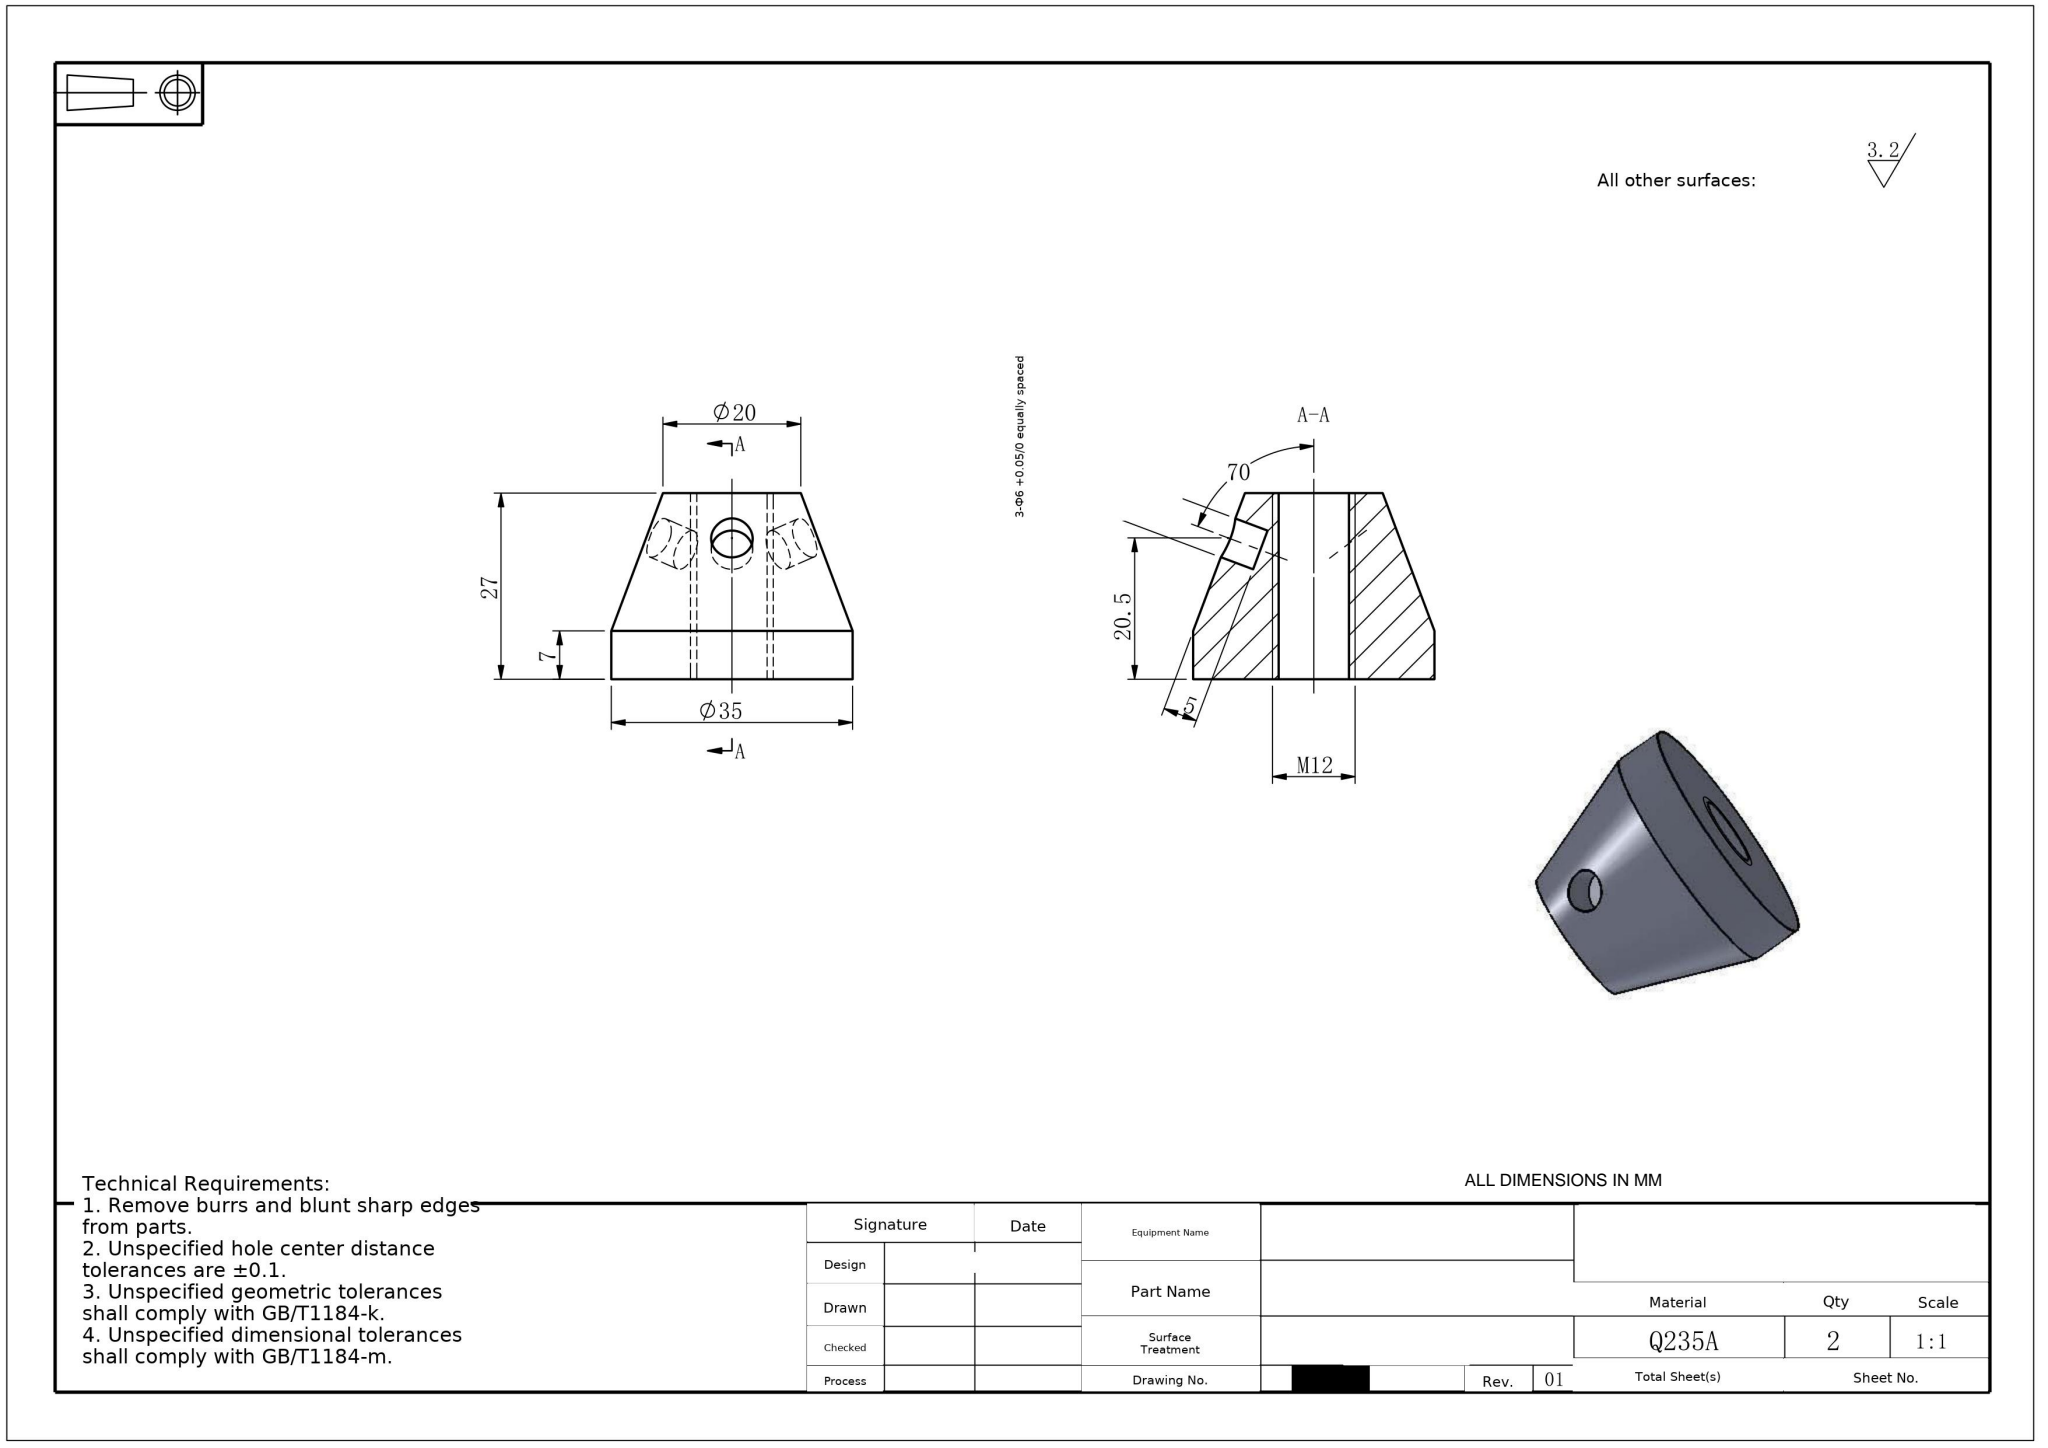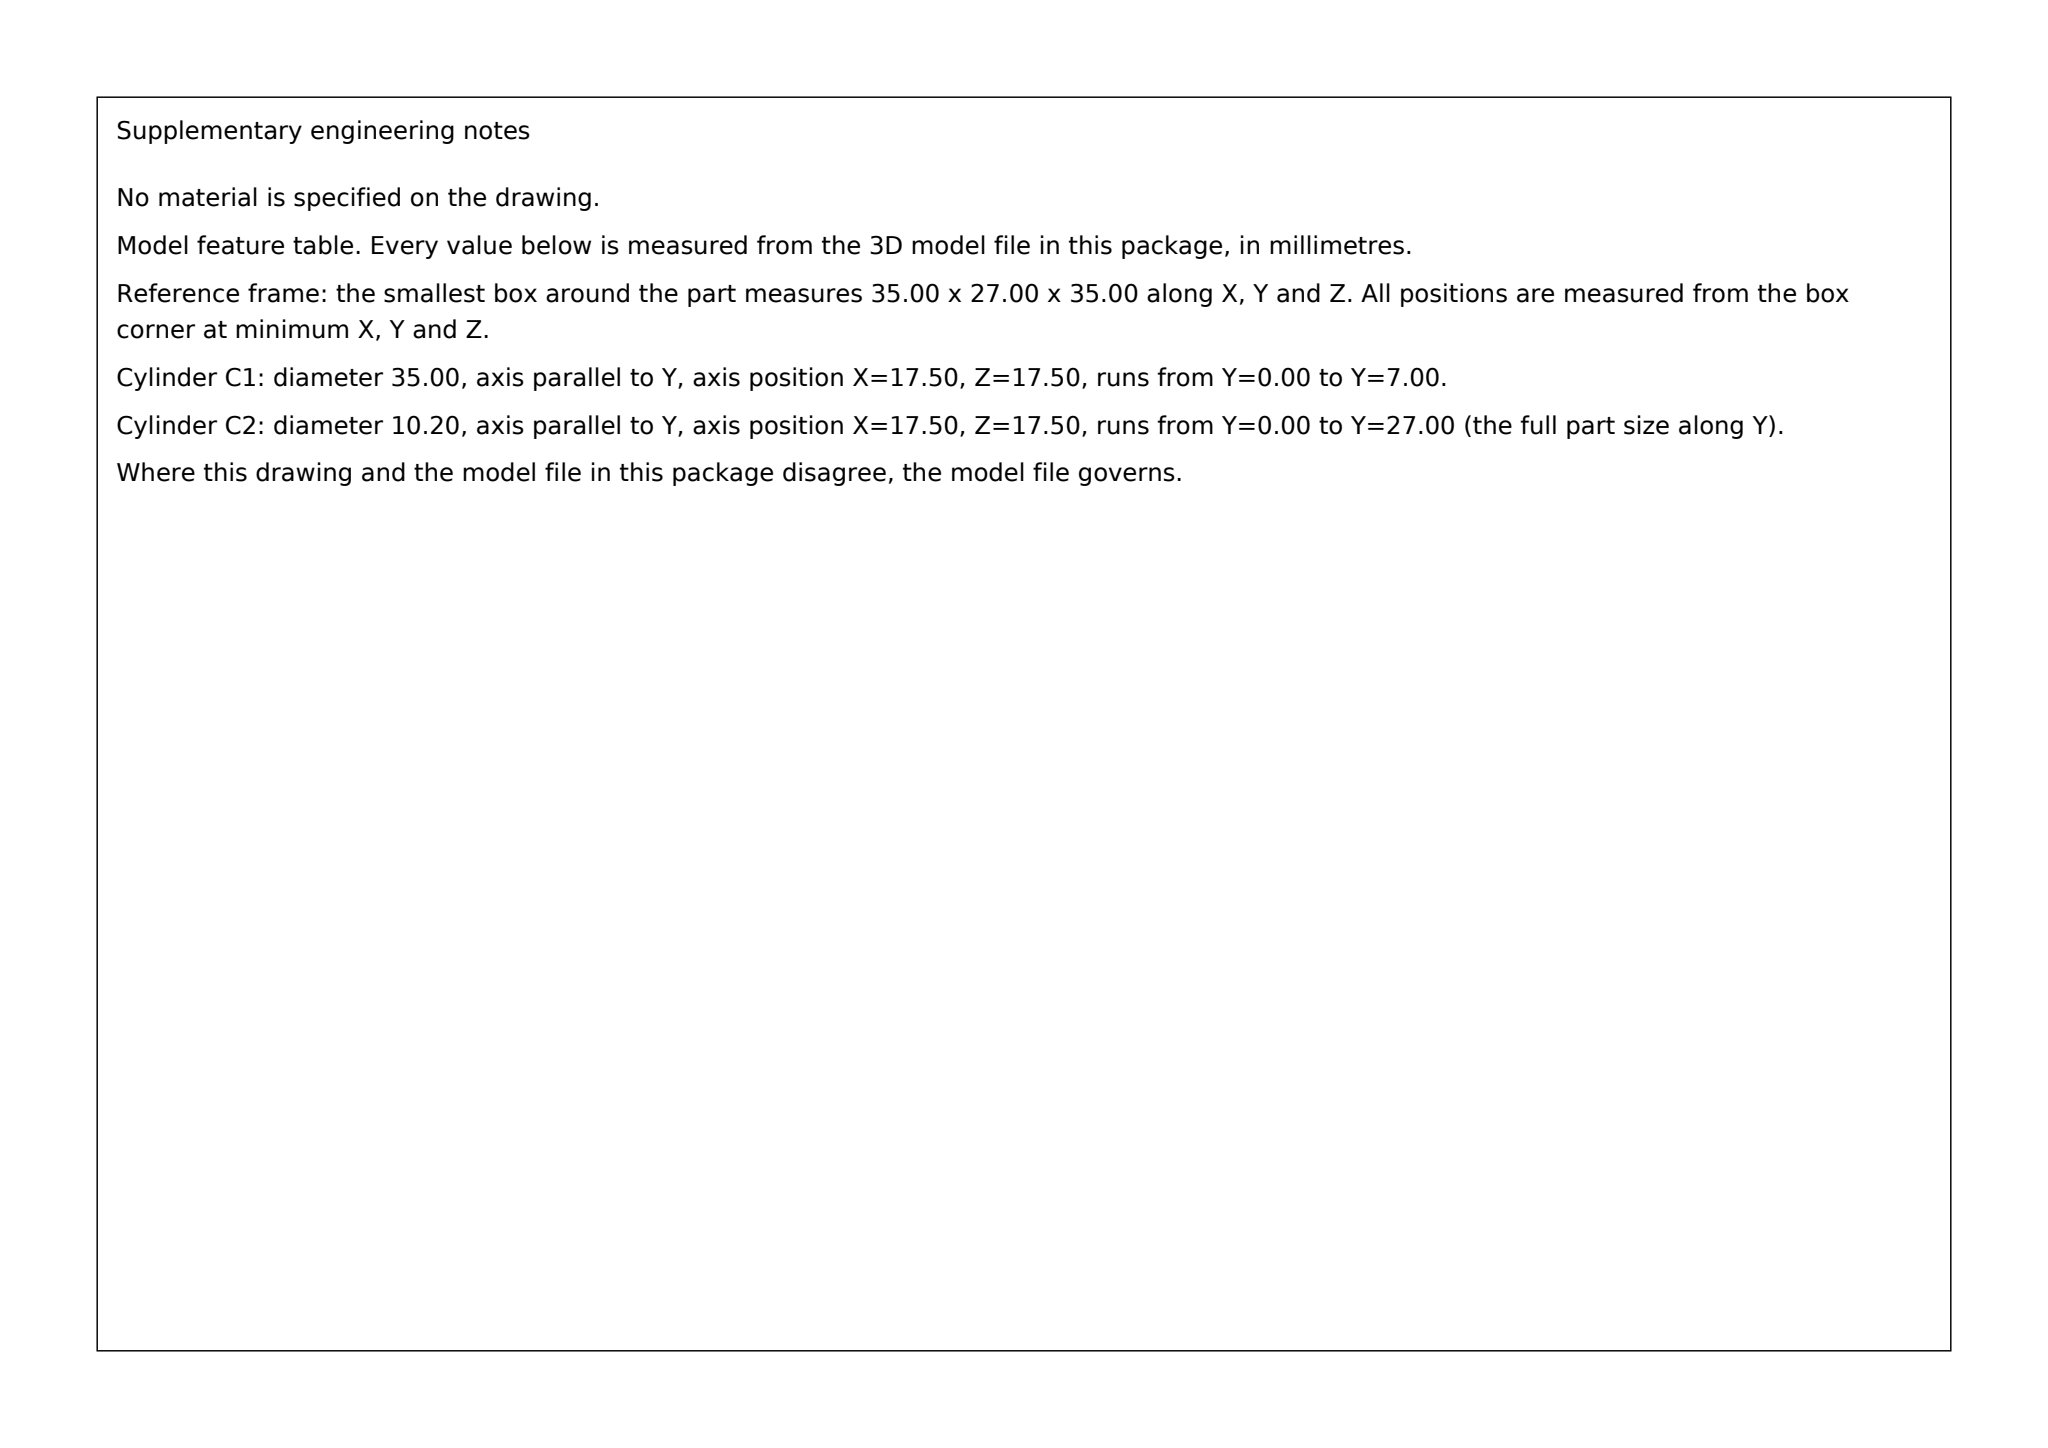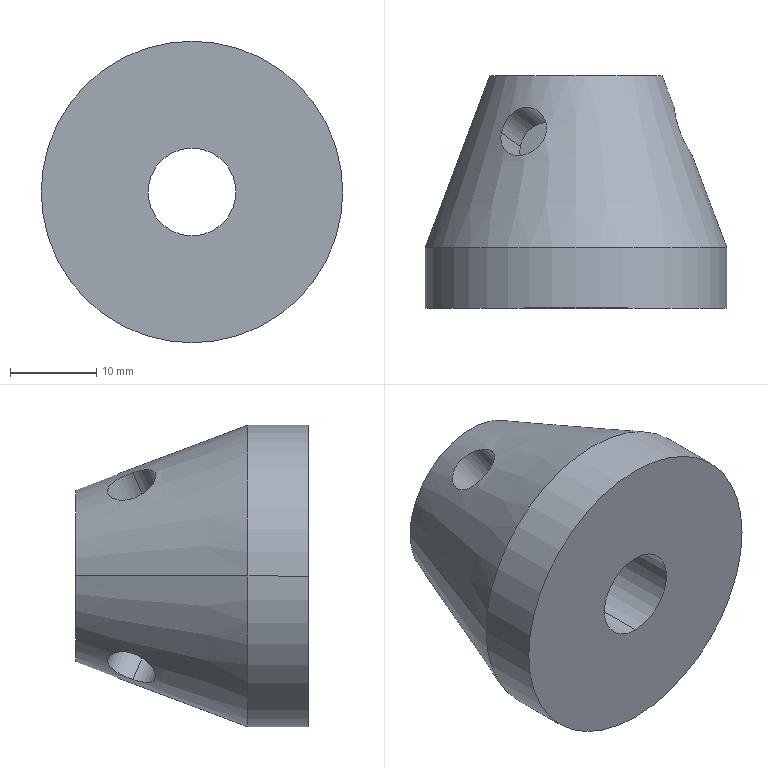Part | SolidWorks | mm | 1 solid | 17 faces | box 35 x 27 x 35 mm | volume 16285 mm3 | cylinder 10 | plane 5 | cone 2 | commonest cylinder face diameters 6 x6 10.2 x2 35 x2
STEP:
#1=CARTESIAN_POINT('',(-48.239,6.094,-8.217));
#2=VERTEX_POINT('',#1);
#3=CARTESIAN_POINT('',(-53.435,6.094,-5.217));
#4=VERTEX_POINT('',#3);
#5=CARTESIAN_POINT('',(-50.837,6.094,-6.717));
#6=DIRECTION('',(-0.4682,0.3511,-0.8109));
#7=DIRECTION('',(0.1756,0.9363,0.3041));
#8=AXIS2_PLACEMENT_3D('',#5,#6,#7);
#9=CIRCLE('',#8,3.);
#10=EDGE_CURVE('',#2,#4,#9,.T.);
#11=ORIENTED_EDGE('',*,*,#10,.F.);
#12=CARTESIAN_POINT('',(-50.42,7.729,-11.993));
#13=VERTEX_POINT('',#12);
#14=CARTESIAN_POINT('',(-48.239,6.094,-8.217));
#15=DIRECTION('',(-0.4682,0.3511,-0.8109));
#16=VECTOR('',#15,1000.);
#17=LINE('',#14,#16);
#18=EDGE_CURVE('',#2,#13,#17,.T.);
#19=ORIENTED_EDGE('',*,*,#18,.T.);
#20=CARTESIAN_POINT('',(-55.616,7.729,-8.993));
#21=VERTEX_POINT('',#20);
#22=CARTESIAN_POINT('',(-55.616,7.729,-8.993));
#23=CARTESIAN_POINT('',(-55.651,7.545,-9.055));
#24=CARTESIAN_POINT('',(-55.672,7.362,-9.13));
#25=CARTESIAN_POINT('',(-55.683,7.01,-9.302));
#26=CARTESIAN_POINT('',(-55.673,6.837,-9.4));
#27=CARTESIAN_POINT('',(-55.622,6.508,-9.614));
#28=CARTESIAN_POINT('',(-55.581,6.354,-9.728));
#29=CARTESIAN_POINT('',(-55.469,6.065,-9.969));
#30=CARTESIAN_POINT('',(-55.397,5.928,-10.097));
#31=CARTESIAN_POINT('',(-55.227,5.685,-10.354));
#32=CARTESIAN_POINT('',(-55.128,5.576,-10.484));
#33=CARTESIAN_POINT('',(-54.902,5.386,-10.746));
#34=CARTESIAN_POINT('',(-54.775,5.304,-10.876));
#35=CARTESIAN_POINT('',(-54.501,5.173,-11.127));
#36=CARTESIAN_POINT('',(-54.352,5.123,-11.25));
#37=CARTESIAN_POINT('',(-54.038,5.057,-11.479));
#38=CARTESIAN_POINT('',(-53.874,5.041,-11.586));
#39=CARTESIAN_POINT('',(-53.533,5.041,-11.782));
#40=CARTESIAN_POINT('',(-53.355,5.058,-11.873));
#41=CARTESIAN_POINT('',(-53.002,5.124,-12.028));
#42=CARTESIAN_POINT('',(-52.824,5.174,-12.096));
#43=CARTESIAN_POINT('',(-52.467,5.306,-12.208));
#44=CARTESIAN_POINT('',(-52.292,5.386,-12.252));
#45=CARTESIAN_POINT('',(-51.955,5.576,-12.316));
#46=CARTESIAN_POINT('',(-51.79,5.686,-12.337));
#47=CARTESIAN_POINT('',(-51.481,5.931,-12.356));
#48=CARTESIAN_POINT('',(-51.338,6.065,-12.355));
#49=CARTESIAN_POINT('',(-51.073,6.354,-12.331));
#50=CARTESIAN_POINT('',(-50.952,6.512,-12.308));
#51=CARTESIAN_POINT('',(-50.743,6.838,-12.246));
#52=CARTESIAN_POINT('',(-50.654,7.008,-12.206));
#53=CARTESIAN_POINT('',(-50.509,7.364,-12.11));
#54=CARTESIAN_POINT('',(-50.455,7.547,-12.055));
#55=CARTESIAN_POINT('',(-50.42,7.729,-11.993));
#56=B_SPLINE_CURVE_WITH_KNOTS('',3,(#22,#23,#24,#25,#26,#27,#28,#29,#30,#31,#32,#33,#34,#35,#36,#37,#38,#39,#40,#41,#42,#43,#44,#45,#46,#47,#48,#49,#50,#51,#52,#53,#54,#55),.UNSPECIFIED.,.F.,.F.,(4,2,2,2,2,2,2,2,2,2,2,2,2,2,2,2,4),(0.01489,0.01548,0.01607,0.01665,0.01724,0.01783,0.01842,0.01901,0.01959,0.02018,0.02077,0.02136,0.02195,0.02253,0.02312,0.02371,0.0243),.UNSPECIFIED.);
#57=EDGE_CURVE('',#21,#13,#56,.T.);
#58=ORIENTED_EDGE('',*,*,#57,.F.);
#59=CARTESIAN_POINT('',(-53.435,6.094,-5.217));
#60=DIRECTION('',(-0.4682,0.3511,-0.8109));
#61=VECTOR('',#60,1000.);
#62=LINE('',#59,#61);
#63=EDGE_CURVE('',#4,#21,#62,.T.);
#64=ORIENTED_EDGE('',*,*,#63,.F.);
#65=EDGE_LOOP('',(#11,#19,#58,#64));
#66=FACE_OUTER_BOUND('',#65,.T.);
#67=CARTESIAN_POINT('',(-50.837,6.094,-6.717));
#68=DIRECTION('',(-0.4682,0.3511,-0.8109));
#69=DIRECTION('',(-0.866,0.,0.5));
#70=AXIS2_PLACEMENT_3D('',#67,#68,#69);
#71=CYLINDRICAL_SURFACE('',#70,3.);
#72=ADVANCED_FACE('',(#66),#71,.F.);
#73=CARTESIAN_POINT('',(-53.435,6.094,5.217));
#74=VERTEX_POINT('',#73);
#75=CARTESIAN_POINT('',(-48.239,6.094,8.217));
#76=VERTEX_POINT('',#75);
#77=CARTESIAN_POINT('',(-50.837,6.094,6.717));
#78=DIRECTION('',(-0.4682,0.3511,0.8109));
#79=DIRECTION('',(0.1756,0.9363,-0.3041));
#80=AXIS2_PLACEMENT_3D('',#77,#78,#79);
#81=CIRCLE('',#80,3.);
#82=EDGE_CURVE('',#74,#76,#81,.T.);
#83=ORIENTED_EDGE('',*,*,#82,.F.);
#84=CARTESIAN_POINT('',(-55.616,7.729,8.993));
#85=VERTEX_POINT('',#84);
#86=CARTESIAN_POINT('',(-53.435,6.094,5.217));
#87=DIRECTION('',(-0.4682,0.3511,0.8109));
#88=VECTOR('',#87,1000.);
#89=LINE('',#86,#88);
#90=EDGE_CURVE('',#74,#85,#89,.T.);
#91=ORIENTED_EDGE('',*,*,#90,.T.);
#92=CARTESIAN_POINT('',(-50.42,7.729,11.993));
#93=VERTEX_POINT('',#92);
#94=CARTESIAN_POINT('',(-50.42,7.729,11.993));
#95=CARTESIAN_POINT('',(-50.455,7.546,12.055));
#96=CARTESIAN_POINT('',(-50.51,7.362,12.111));
#97=CARTESIAN_POINT('',(-50.654,7.009,12.206));
#98=CARTESIAN_POINT('',(-50.743,6.838,12.246));
#99=CARTESIAN_POINT('',(-50.954,6.508,12.309));
#100=CARTESIAN_POINT('',(-51.074,6.353,12.331));
#101=CARTESIAN_POINT('',(-51.338,6.064,12.355));
#102=CARTESIAN_POINT('',(-51.484,5.928,12.356));
#103=CARTESIAN_POINT('',(-51.794,5.684,12.337));
#104=CARTESIAN_POINT('',(-51.956,5.576,12.316));
#105=CARTESIAN_POINT('',(-52.294,5.386,12.252));
#106=CARTESIAN_POINT('',(-52.471,5.304,12.207));
#107=CARTESIAN_POINT('',(-52.824,5.174,12.095));
#108=CARTESIAN_POINT('',(-53.002,5.124,12.028));
#109=CARTESIAN_POINT('',(-53.358,5.057,11.871));
#110=CARTESIAN_POINT('',(-53.535,5.041,11.781));
#111=CARTESIAN_POINT('',(-53.874,5.041,11.585));
#112=CARTESIAN_POINT('',(-54.04,5.057,11.478));
#113=CARTESIAN_POINT('',(-54.355,5.124,11.247));
#114=CARTESIAN_POINT('',(-54.502,5.174,11.127));
#115=CARTESIAN_POINT('',(-54.775,5.304,10.876));
#116=CARTESIAN_POINT('',(-54.902,5.386,10.745));
#117=CARTESIAN_POINT('',(-55.128,5.576,10.485));
#118=CARTESIAN_POINT('',(-55.227,5.684,10.355));
#119=CARTESIAN_POINT('',(-55.398,5.929,10.096));
#120=CARTESIAN_POINT('',(-55.469,6.065,9.969));
#121=CARTESIAN_POINT('',(-55.581,6.354,9.729));
#122=CARTESIAN_POINT('',(-55.622,6.508,9.614));
#123=CARTESIAN_POINT('',(-55.673,6.839,9.399));
#124=CARTESIAN_POINT('',(-55.683,7.009,9.302));
#125=CARTESIAN_POINT('',(-55.672,7.361,9.131));
#126=CARTESIAN_POINT('',(-55.651,7.545,9.055));
#127=CARTESIAN_POINT('',(-55.616,7.729,8.993));
#128=B_SPLINE_CURVE_WITH_KNOTS('',3,(#94,#95,#96,#97,#98,#99,#100,#101,#102,#103,#104,#105,#106,#107,#108,#109,#110,#111,#112,#113,#114,#115,#116,#117,#118,#119,#120,#121,#122,#123,#124,#125,#126,#127),.UNSPECIFIED.,.F.,.F.,(4,2,2,2,2,2,2,2,2,2,2,2,2,2,2,2,4),(0.008823,0.009411,0.009999,0.01059,0.01117,0.01176,0.01235,0.01294,0.01353,0.01411,0.0147,0.01529,0.01588,0.01647,0.01705,0.01764,0.01823),.UNSPECIFIED.);
#129=EDGE_CURVE('',#93,#85,#128,.T.);
#130=ORIENTED_EDGE('',*,*,#129,.F.);
#131=CARTESIAN_POINT('',(-48.239,6.094,8.217));
#132=DIRECTION('',(-0.4682,0.3511,0.8109));
#133=VECTOR('',#132,1000.);
#134=LINE('',#131,#133);
#135=EDGE_CURVE('',#76,#93,#134,.T.);
#136=ORIENTED_EDGE('',*,*,#135,.F.);
#137=EDGE_LOOP('',(#83,#91,#130,#136));
#138=FACE_OUTER_BOUND('',#137,.T.);
#139=CARTESIAN_POINT('',(-50.837,6.094,6.717));
#140=DIRECTION('',(-0.4682,0.3511,0.8109));
#141=DIRECTION('',(0.866,0.,0.5));
#142=AXIS2_PLACEMENT_3D('',#139,#140,#141);
#143=CYLINDRICAL_SURFACE('',#142,3.);
#144=ADVANCED_FACE('',(#138),#143,.F.);
#145=CARTESIAN_POINT('',(-38.15,3.285,0.));
#146=VERTEX_POINT('',#145);
#147=CARTESIAN_POINT('',(-40.257,8.903,0.));
#148=VERTEX_POINT('',#147);
#149=CARTESIAN_POINT('',(-39.203,6.094,0.));
#150=DIRECTION('',(0.9363,0.3511,-0.));
#151=DIRECTION('',(-0.3511,0.9363,0.));
#152=AXIS2_PLACEMENT_3D('',#149,#150,#151);
#153=CIRCLE('',#152,3.);
#154=EDGE_CURVE('',#146,#148,#153,.T.);
#155=ORIENTED_EDGE('',*,*,#154,.F.);
#156=CARTESIAN_POINT('',(-33.468,5.041,0.));
#157=VERTEX_POINT('',#156);
#158=CARTESIAN_POINT('',(-38.15,3.285,0.));
#159=DIRECTION('',(0.9363,0.3511,-0.));
#160=VECTOR('',#159,1000.);
#161=LINE('',#158,#160);
#162=EDGE_CURVE('',#146,#157,#161,.T.);
#163=ORIENTED_EDGE('',*,*,#162,.T.);
#164=CARTESIAN_POINT('',(-35.575,10.659,0.));
#165=VERTEX_POINT('',#164);
#166=CARTESIAN_POINT('',(-35.575,10.659,0.));
#167=CARTESIAN_POINT('',(-35.575,10.659,-0.1967));
#168=CARTESIAN_POINT('',(-35.573,10.639,-0.3918));
#169=CARTESIAN_POINT('',(-35.563,10.56,-0.7784));
#170=CARTESIAN_POINT('',(-35.556,10.501,-0.969));
#171=CARTESIAN_POINT('',(-35.535,10.349,-1.33));
#172=CARTESIAN_POINT('',(-35.521,10.255,-1.503));
#173=CARTESIAN_POINT('',(-35.485,10.035,-1.831));
#174=CARTESIAN_POINT('',(-35.463,9.911,-1.982));
#175=CARTESIAN_POINT('',(-35.41,9.637,-2.258));
#176=CARTESIAN_POINT('',(-35.377,9.485,-2.384));
#177=CARTESIAN_POINT('',(-35.302,9.166,-2.602));
#178=CARTESIAN_POINT('',(-35.258,8.998,-2.694));
#179=CARTESIAN_POINT('',(-35.159,8.648,-2.845));
#180=CARTESIAN_POINT('',(-35.103,8.465,-2.903));
#181=CARTESIAN_POINT('',(-34.981,8.1,-2.98));
#182=CARTESIAN_POINT('',(-34.915,7.917,-3.));
#183=CARTESIAN_POINT('',(-34.772,7.547,-3.));
#184=CARTESIAN_POINT('',(-34.697,7.365,-2.981));
#185=CARTESIAN_POINT('',(-34.543,7.012,-2.904));
#186=CARTESIAN_POINT('',(-34.462,6.839,-2.847));
#187=CARTESIAN_POINT('',(-34.303,6.51,-2.696));
#188=CARTESIAN_POINT('',(-34.225,6.356,-2.604));
#189=CARTESIAN_POINT('',(-34.071,6.066,-2.387));
#190=CARTESIAN_POINT('',(-33.996,5.93,-2.26));
#191=CARTESIAN_POINT('',(-33.859,5.685,-1.984));
#192=CARTESIAN_POINT('',(-33.795,5.575,-1.831));
#193=CARTESIAN_POINT('',(-33.681,5.384,-1.503));
#194=CARTESIAN_POINT('',(-33.632,5.304,-1.331));
#195=CARTESIAN_POINT('',(-33.552,5.174,-0.9692));
#196=CARTESIAN_POINT('',(-33.521,5.124,-0.7778));
#197=CARTESIAN_POINT('',(-33.479,5.057,-0.3924));
#198=CARTESIAN_POINT('',(-33.468,5.041,-0.1974));
#199=CARTESIAN_POINT('',(-33.468,5.041,0.));
#200=B_SPLINE_CURVE_WITH_KNOTS('',3,(#166,#167,#168,#169,#170,#171,#172,#173,#174,#175,#176,#177,#178,#179,#180,#181,#182,#183,#184,#185,#186,#187,#188,#189,#190,#191,#192,#193,#194,#195,#196,#197,#198,#199),.UNSPECIFIED.,.F.,.F.,(4,2,2,2,2,2,2,2,2,2,2,2,2,2,2,2,4),(0.01126,0.01185,0.01244,0.01303,0.01362,0.01421,0.01479,0.01538,0.01597,0.01656,0.01715,0.01773,0.01832,0.01891,0.0195,0.02009,0.02068),.UNSPECIFIED.);
#201=EDGE_CURVE('',#165,#157,#200,.T.);
#202=ORIENTED_EDGE('',*,*,#201,.F.);
#203=CARTESIAN_POINT('',(-40.257,8.903,0.));
#204=DIRECTION('',(0.9363,0.3511,-0.));
#205=VECTOR('',#204,1000.);
#206=LINE('',#203,#205);
#207=EDGE_CURVE('',#148,#165,#206,.T.);
#208=ORIENTED_EDGE('',*,*,#207,.F.);
#209=EDGE_LOOP('',(#155,#163,#202,#208));
#210=FACE_OUTER_BOUND('',#209,.T.);
#211=CARTESIAN_POINT('',(-39.203,6.094,0.));
#212=DIRECTION('',(0.9363,0.3511,-0.));
#213=DIRECTION('',(-0.3511,0.9363,0.));
#214=AXIS2_PLACEMENT_3D('',#211,#212,#213);
#215=CYLINDRICAL_SURFACE('',#214,3.);
#216=ADVANCED_FACE('',(#210),#215,.F.);
#217=CARTESIAN_POINT('',(-46.959,14.35,5.1));
#218=VERTEX_POINT('',#217);
#219=CARTESIAN_POINT('',(-46.959,14.35,-5.1));
#220=VERTEX_POINT('',#219);
#221=CARTESIAN_POINT('',(-46.959,14.35,0.));
#222=DIRECTION('',(0.,-1.,0.));
#223=DIRECTION('',(0.,0.,-1.));
#224=AXIS2_PLACEMENT_3D('',#221,#222,#223);
#225=CIRCLE('',#224,5.1);
#226=EDGE_CURVE('',#218,#220,#225,.T.);
#227=ORIENTED_EDGE('',*,*,#226,.F.);
#228=CARTESIAN_POINT('',(-46.959,-12.65,5.1));
#229=VERTEX_POINT('',#228);
#230=CARTESIAN_POINT('',(-46.959,-12.65,5.1));
#231=DIRECTION('',(0.,-1.,0.));
#232=VECTOR('',#231,1000.);
#233=LINE('',#230,#232);
#234=EDGE_CURVE('',#218,#229,#233,.T.);
#235=ORIENTED_EDGE('',*,*,#234,.T.);
#236=CARTESIAN_POINT('',(-46.959,-12.65,-5.1));
#237=VERTEX_POINT('',#236);
#238=CARTESIAN_POINT('',(-46.959,-12.65,0.));
#239=DIRECTION('',(0.,-1.,0.));
#240=DIRECTION('',(0.,0.,-1.));
#241=AXIS2_PLACEMENT_3D('',#238,#239,#240);
#242=CIRCLE('',#241,5.1);
#243=EDGE_CURVE('',#229,#237,#242,.T.);
#244=ORIENTED_EDGE('',*,*,#243,.T.);
#245=CARTESIAN_POINT('',(-46.959,-12.65,-5.1));
#246=DIRECTION('',(0.,-1.,0.));
#247=VECTOR('',#246,1000.);
#248=LINE('',#245,#247);
#249=EDGE_CURVE('',#220,#237,#248,.T.);
#250=ORIENTED_EDGE('',*,*,#249,.F.);
#251=EDGE_LOOP('',(#227,#235,#244,#250));
#252=FACE_OUTER_BOUND('',#251,.T.);
#253=CARTESIAN_POINT('',(-46.959,-12.65,0.));
#254=DIRECTION('',(0.,-1.,0.));
#255=DIRECTION('',(0.,0.,-1.));
#256=AXIS2_PLACEMENT_3D('',#253,#254,#255);
#257=CYLINDRICAL_SURFACE('',#256,5.1);
#258=ADVANCED_FACE('',(#252),#257,.F.);
#259=CARTESIAN_POINT('',(-64.459,-12.65,0.));
#260=VERTEX_POINT('',#259);
#261=CARTESIAN_POINT('',(-29.459,-12.65,0.));
#262=VERTEX_POINT('',#261);
#263=CARTESIAN_POINT('',(-46.959,-12.65,0.));
#264=DIRECTION('',(0.,1.,0.));
#265=DIRECTION('',(-1.,0.,0.));
#266=AXIS2_PLACEMENT_3D('',#263,#264,#265);
#267=CIRCLE('',#266,17.5);
#268=EDGE_CURVE('',#260,#262,#267,.T.);
#269=ORIENTED_EDGE('',*,*,#268,.T.);
#270=CARTESIAN_POINT('',(-29.459,-5.65,0.));
#271=VERTEX_POINT('',#270);
#272=CARTESIAN_POINT('',(-29.459,14.35,0.));
#273=DIRECTION('',(0.,1.,0.));
#274=VECTOR('',#273,1000.);
#275=LINE('',#272,#274);
#276=EDGE_CURVE('',#262,#271,#275,.T.);
#277=ORIENTED_EDGE('',*,*,#276,.T.);
#278=CARTESIAN_POINT('',(-64.459,-5.65,0.));
#279=VERTEX_POINT('',#278);
#280=CARTESIAN_POINT('',(-46.959,-5.65,0.));
#281=DIRECTION('',(0.,1.,0.));
#282=DIRECTION('',(-1.,0.,0.));
#283=AXIS2_PLACEMENT_3D('',#280,#281,#282);
#284=CIRCLE('',#283,17.5);
#285=EDGE_CURVE('',#279,#271,#284,.T.);
#286=ORIENTED_EDGE('',*,*,#285,.F.);
#287=CARTESIAN_POINT('',(-64.459,14.35,0.));
#288=DIRECTION('',(0.,1.,0.));
#289=VECTOR('',#288,1000.);
#290=LINE('',#287,#289);
#291=EDGE_CURVE('',#260,#279,#290,.T.);
#292=ORIENTED_EDGE('',*,*,#291,.F.);
#293=EDGE_LOOP('',(#269,#277,#286,#292));
#294=FACE_OUTER_BOUND('',#293,.T.);
#295=CARTESIAN_POINT('',(-46.959,14.35,0.));
#296=DIRECTION('',(0.,1.,0.));
#297=DIRECTION('',(-1.,0.,0.));
#298=AXIS2_PLACEMENT_3D('',#295,#296,#297);
#299=CYLINDRICAL_SURFACE('',#298,17.5);
#300=ADVANCED_FACE('',(#294),#299,.T.);
#301=ORIENTED_EDGE('',*,*,#129,.T.);
#302=CARTESIAN_POINT('',(-55.616,7.729,8.993));
#303=CARTESIAN_POINT('',(-55.544,8.098,8.87));
#304=CARTESIAN_POINT('',(-55.413,8.474,8.802));
#305=CARTESIAN_POINT('',(-55.144,8.997,8.786));
#306=CARTESIAN_POINT('',(-55.04,9.167,8.795));
#307=CARTESIAN_POINT('',(-54.813,9.487,8.839));
#308=CARTESIAN_POINT('',(-54.69,9.636,8.873));
#309=CARTESIAN_POINT('',(-54.423,9.911,8.965));
#310=CARTESIAN_POINT('',(-54.279,10.037,9.022));
#311=CARTESIAN_POINT('',(-53.98,10.255,9.154));
#312=CARTESIAN_POINT('',(-53.825,10.349,9.228));
#313=CARTESIAN_POINT('',(-53.335,10.579,9.474));
#314=CARTESIAN_POINT('',(-52.993,10.659,9.662));
#315=CARTESIAN_POINT('',(-52.478,10.658,9.959));
#316=CARTESIAN_POINT('',(-52.31,10.638,10.058));
#317=CARTESIAN_POINT('',(-51.982,10.56,10.259));
#318=CARTESIAN_POINT('',(-51.82,10.501,10.361));
#319=CARTESIAN_POINT('',(-51.517,10.348,10.561));
#320=CARTESIAN_POINT('',(-51.375,10.254,10.658));
#321=CARTESIAN_POINT('',(-51.11,10.034,10.853));
#322=CARTESIAN_POINT('',(-50.989,9.909,10.948));
#323=CARTESIAN_POINT('',(-50.777,9.634,11.132));
#324=CARTESIAN_POINT('',(-50.685,9.484,11.223));
#325=CARTESIAN_POINT('',(-50.533,9.163,11.398));
#326=CARTESIAN_POINT('',(-50.475,8.995,11.482));
#327=CARTESIAN_POINT('',(-50.395,8.646,11.643));
#328=CARTESIAN_POINT('',(-50.373,8.463,11.72));
#329=CARTESIAN_POINT('',(-50.368,8.097,11.865));
#330=CARTESIAN_POINT('',(-50.384,7.913,11.932));
#331=CARTESIAN_POINT('',(-50.42,7.729,11.993));
#332=B_SPLINE_CURVE_WITH_KNOTS('',3,(#302,#303,#304,#305,#306,#307,#308,#309,#310,#311,#312,#313,#314,#315,#316,#317,#318,#319,#320,#321,#322,#323,#324,#325,#326,#327,#328,#329,#330,#331),.UNSPECIFIED.,.F.,.F.,(4,2,2,2,2,2,2,2,2,2,2,2,2,2,4),(0.01823,0.0194,0.01999,0.02058,0.02117,0.02176,0.02293,0.02352,0.02411,0.0247,0.02529,0.02587,0.02646,0.02705,0.02764),.UNSPECIFIED.);
#333=EDGE_CURVE('',#85,#93,#332,.T.);
#334=ORIENTED_EDGE('',*,*,#333,.T.);
#335=EDGE_LOOP('',(#301,#334));
#336=FACE_BOUND('',#335,.T.);
#337=CARTESIAN_POINT('',(-56.959,14.35,0.));
#338=VERTEX_POINT('',#337);
#339=CARTESIAN_POINT('',(-36.959,14.35,0.));
#340=VERTEX_POINT('',#339);
#341=CARTESIAN_POINT('',(-46.959,14.35,0.));
#342=DIRECTION('',(0.,1.,0.));
#343=DIRECTION('',(-1.,0.,0.));
#344=AXIS2_PLACEMENT_3D('',#341,#342,#343);
#345=CIRCLE('',#344,10.);
#346=EDGE_CURVE('',#338,#340,#345,.T.);
#347=ORIENTED_EDGE('',*,*,#346,.F.);
#348=CARTESIAN_POINT('',(-64.459,-5.65,0.));
#349=DIRECTION('',(-0.3511,-0.9363,0.));
#350=VECTOR('',#349,1000.);
#351=LINE('',#348,#350);
#352=EDGE_CURVE('',#338,#279,#351,.T.);
#353=ORIENTED_EDGE('',*,*,#352,.T.);
#354=ORIENTED_EDGE('',*,*,#285,.T.);
#355=CARTESIAN_POINT('',(-29.459,-5.65,0.));
#356=DIRECTION('',(0.3511,-0.9363,0.));
#357=VECTOR('',#356,1000.);
#358=LINE('',#355,#357);
#359=EDGE_CURVE('',#157,#271,#358,.T.);
#360=ORIENTED_EDGE('',*,*,#359,.F.);
#361=CARTESIAN_POINT('',(-33.468,5.041,0.));
#362=CARTESIAN_POINT('',(-33.468,5.041,0.1974));
#363=CARTESIAN_POINT('',(-33.479,5.058,0.3959));
#364=CARTESIAN_POINT('',(-33.521,5.124,0.7802));
#365=CARTESIAN_POINT('',(-33.552,5.174,0.9689));
#366=CARTESIAN_POINT('',(-33.633,5.305,1.334));
#367=CARTESIAN_POINT('',(-33.682,5.386,1.507));
#368=CARTESIAN_POINT('',(-33.795,5.576,1.831));
#369=CARTESIAN_POINT('',(-33.859,5.687,1.985));
#370=CARTESIAN_POINT('',(-33.997,5.931,2.261));
#371=CARTESIAN_POINT('',(-34.07,6.064,2.385));
#372=CARTESIAN_POINT('',(-34.224,6.355,2.603));
#373=CARTESIAN_POINT('',(-34.304,6.512,2.697));
#374=CARTESIAN_POINT('',(-34.462,6.838,2.846));
#375=CARTESIAN_POINT('',(-34.541,7.008,2.903));
#376=CARTESIAN_POINT('',(-34.697,7.365,2.981));
#377=CARTESIAN_POINT('',(-34.772,7.547,3.));
#378=CARTESIAN_POINT('',(-34.913,7.912,3.));
#379=CARTESIAN_POINT('',(-34.98,8.099,2.98));
#380=CARTESIAN_POINT('',(-35.103,8.466,2.903));
#381=CARTESIAN_POINT('',(-35.158,8.646,2.846));
#382=CARTESIAN_POINT('',(-35.258,8.995,2.696));
#383=CARTESIAN_POINT('',(-35.302,9.167,2.601));
#384=CARTESIAN_POINT('',(-35.377,9.485,2.384));
#385=CARTESIAN_POINT('',(-35.409,9.634,2.26));
#386=CARTESIAN_POINT('',(-35.491,10.049,1.843));
#387=CARTESIAN_POINT('',(-35.524,10.272,1.514));
#388=CARTESIAN_POINT('',(-35.556,10.502,0.9677));
#389=CARTESIAN_POINT('',(-35.563,10.56,0.7805));
#390=CARTESIAN_POINT('',(-35.573,10.638,0.3962));
#391=CARTESIAN_POINT('',(-35.575,10.659,0.1967));
#392=CARTESIAN_POINT('',(-35.575,10.659,0.));
#393=B_SPLINE_CURVE_WITH_KNOTS('',3,(#361,#362,#363,#364,#365,#366,#367,#368,#369,#370,#371,#372,#373,#374,#375,#376,#377,#378,#379,#380,#381,#382,#383,#384,#385,#386,#387,#388,#389,#390,#391,#392),.UNSPECIFIED.,.F.,.F.,(4,2,2,2,2,2,2,2,2,2,2,2,2,2,2,4),(0.001855,0.002443,0.003031,0.003619,0.004207,0.004796,0.005384,0.005972,0.00656,0.007148,0.007736,0.008324,0.008912,0.01009,0.01068,0.01126),.UNSPECIFIED.);
#394=EDGE_CURVE('',#157,#165,#393,.T.);
#395=ORIENTED_EDGE('',*,*,#394,.T.);
#396=CARTESIAN_POINT('',(-29.459,-5.65,0.));
#397=DIRECTION('',(0.3511,-0.9363,0.));
#398=VECTOR('',#397,1000.);
#399=LINE('',#396,#398);
#400=EDGE_CURVE('',#340,#165,#399,.T.);
#401=ORIENTED_EDGE('',*,*,#400,.F.);
#402=EDGE_LOOP('',(#347,#353,#354,#360,#395,#401));
#403=FACE_OUTER_BOUND('',#402,.T.);
#404=CARTESIAN_POINT('',(-46.959,-5.65,0.));
#405=DIRECTION('',(-0.,-1.,0.));
#406=DIRECTION('',(1.,-0.,0.));
#407=AXIS2_PLACEMENT_3D('',#404,#405,#406);
#408=CONICAL_SURFACE('',#407,17.5,0.3588);
#409=ADVANCED_FACE('',(#336,#403),#408,.T.);
#410=CARTESIAN_POINT('',(-46.959,14.35,0.));
#411=DIRECTION('',(0.,-1.,0.));
#412=DIRECTION('',(0.,0.,-1.));
#413=AXIS2_PLACEMENT_3D('',#410,#411,#412);
#414=CIRCLE('',#413,5.1);
#415=EDGE_CURVE('',#220,#218,#414,.T.);
#416=ORIENTED_EDGE('',*,*,#415,.T.);
#417=ORIENTED_EDGE('',*,*,#226,.T.);
#418=EDGE_LOOP('',(#416,#417));
#419=FACE_BOUND('',#418,.T.);
#420=CARTESIAN_POINT('',(-46.959,14.35,0.));
#421=DIRECTION('',(0.,1.,0.));
#422=DIRECTION('',(-1.,0.,0.));
#423=AXIS2_PLACEMENT_3D('',#420,#421,#422);
#424=CIRCLE('',#423,10.);
#425=EDGE_CURVE('',#340,#338,#424,.T.);
#426=ORIENTED_EDGE('',*,*,#425,.T.);
#427=ORIENTED_EDGE('',*,*,#346,.T.);
#428=EDGE_LOOP('',(#426,#427));
#429=FACE_OUTER_BOUND('',#428,.T.);
#430=CARTESIAN_POINT('',(-46.959,14.35,0.));
#431=DIRECTION('',(-0.,-1.,0.));
#432=DIRECTION('',(1.,-0.,0.));
#433=AXIS2_PLACEMENT_3D('',#430,#431,#432);
#434=PLANE('',#433);
#435=ADVANCED_FACE('',(#419,#429),#434,.F.);
#436=ORIENTED_EDGE('',*,*,#352,.F.);
#437=ORIENTED_EDGE('',*,*,#425,.F.);
#438=ORIENTED_EDGE('',*,*,#400,.T.);
#439=ORIENTED_EDGE('',*,*,#201,.T.);
#440=ORIENTED_EDGE('',*,*,#359,.T.);
#441=CARTESIAN_POINT('',(-46.959,-5.65,0.));
#442=DIRECTION('',(0.,1.,0.));
#443=DIRECTION('',(-1.,0.,0.));
#444=AXIS2_PLACEMENT_3D('',#441,#442,#443);
#445=CIRCLE('',#444,17.5);
#446=EDGE_CURVE('',#271,#279,#445,.T.);
#447=ORIENTED_EDGE('',*,*,#446,.T.);
#448=EDGE_LOOP('',(#436,#437,#438,#439,#440,#447));
#449=FACE_OUTER_BOUND('',#448,.T.);
#450=ORIENTED_EDGE('',*,*,#57,.T.);
#451=CARTESIAN_POINT('',(-50.42,7.729,-11.993));
#452=CARTESIAN_POINT('',(-50.384,7.912,-11.932));
#453=CARTESIAN_POINT('',(-50.367,8.098,-11.865));
#454=CARTESIAN_POINT('',(-50.373,8.466,-11.719));
#455=CARTESIAN_POINT('',(-50.395,8.646,-11.643));
#456=CARTESIAN_POINT('',(-50.475,8.995,-11.482));
#457=CARTESIAN_POINT('',(-50.535,9.167,-11.396));
#458=CARTESIAN_POINT('',(-50.686,9.485,-11.222));
#459=CARTESIAN_POINT('',(-50.777,9.634,-11.132));
#460=CARTESIAN_POINT('',(-50.99,9.91,-10.947));
#461=CARTESIAN_POINT('',(-51.112,10.036,-10.851));
#462=CARTESIAN_POINT('',(-51.375,10.254,-10.658));
#463=CARTESIAN_POINT('',(-51.518,10.348,-10.56));
#464=CARTESIAN_POINT('',(-51.824,10.502,-10.359));
#465=CARTESIAN_POINT('',(-51.982,10.56,-10.259));
#466=CARTESIAN_POINT('',(-52.31,10.638,-10.058));
#467=CARTESIAN_POINT('',(-52.481,10.659,-9.957));
#468=CARTESIAN_POINT('',(-52.823,10.659,-9.76));
#469=CARTESIAN_POINT('',(-52.993,10.639,-9.664));
#470=CARTESIAN_POINT('',(-53.332,10.56,-9.48));
#471=CARTESIAN_POINT('',(-53.501,10.501,-9.39));
#472=CARTESIAN_POINT('',(-53.987,10.272,-9.147));
#473=CARTESIAN_POINT('',(-54.292,10.046,-9.01));
#474=CARTESIAN_POINT('',(-54.691,9.635,-8.873));
#475=CARTESIAN_POINT('',(-54.816,9.484,-8.838));
#476=CARTESIAN_POINT('',(-55.043,9.163,-8.795));
#477=CARTESIAN_POINT('',(-55.144,8.996,-8.786));
#478=CARTESIAN_POINT('',(-55.324,8.646,-8.797));
#479=CARTESIAN_POINT('',(-55.403,8.463,-8.817));
#480=CARTESIAN_POINT('',(-55.53,8.097,-8.884));
#481=CARTESIAN_POINT('',(-55.58,7.914,-8.932));
#482=CARTESIAN_POINT('',(-55.616,7.729,-8.993));
#483=B_SPLINE_CURVE_WITH_KNOTS('',3,(#451,#452,#453,#454,#455,#456,#457,#458,#459,#460,#461,#462,#463,#464,#465,#466,#467,#468,#469,#470,#471,#472,#473,#474,#475,#476,#477,#478,#479,#480,#481,#482),.UNSPECIFIED.,.F.,.F.,(4,2,2,2,2,2,2,2,2,2,2,2,2,2,2,4),(0.005477,0.006066,0.006654,0.007242,0.007831,0.008419,0.009007,0.009596,0.01018,0.01077,0.01136,0.01254,0.01313,0.01371,0.0143,0.01489),.UNSPECIFIED.);
#484=EDGE_CURVE('',#13,#21,#483,.T.);
#485=ORIENTED_EDGE('',*,*,#484,.T.);
#486=EDGE_LOOP('',(#450,#485));
#487=FACE_BOUND('',#486,.T.);
#488=CARTESIAN_POINT('',(-46.959,-5.65,0.));
#489=DIRECTION('',(-0.,-1.,0.));
#490=DIRECTION('',(1.,-0.,0.));
#491=AXIS2_PLACEMENT_3D('',#488,#489,#490);
#492=CONICAL_SURFACE('',#491,17.5,0.3588);
#493=ADVANCED_FACE('',(#449,#487),#492,.T.);
#494=ORIENTED_EDGE('',*,*,#276,.F.);
#495=CARTESIAN_POINT('',(-46.959,-12.65,0.));
#496=DIRECTION('',(0.,1.,0.));
#497=DIRECTION('',(-1.,0.,0.));
#498=AXIS2_PLACEMENT_3D('',#495,#496,#497);
#499=CIRCLE('',#498,17.5);
#500=EDGE_CURVE('',#262,#260,#499,.T.);
#501=ORIENTED_EDGE('',*,*,#500,.T.);
#502=ORIENTED_EDGE('',*,*,#291,.T.);
#503=ORIENTED_EDGE('',*,*,#446,.F.);
#504=EDGE_LOOP('',(#494,#501,#502,#503));
#505=FACE_OUTER_BOUND('',#504,.T.);
#506=CARTESIAN_POINT('',(-46.959,14.35,0.));
#507=DIRECTION('',(0.,1.,0.));
#508=DIRECTION('',(-1.,0.,0.));
#509=AXIS2_PLACEMENT_3D('',#506,#507,#508);
#510=CYLINDRICAL_SURFACE('',#509,17.5);
#511=ADVANCED_FACE('',(#505),#510,.T.);
#512=CARTESIAN_POINT('',(-46.959,-12.65,0.));
#513=DIRECTION('',(0.,-1.,0.));
#514=DIRECTION('',(0.,0.,-1.));
#515=AXIS2_PLACEMENT_3D('',#512,#513,#514);
#516=CIRCLE('',#515,5.1);
#517=EDGE_CURVE('',#237,#229,#516,.T.);
#518=ORIENTED_EDGE('',*,*,#517,.F.);
#519=ORIENTED_EDGE('',*,*,#243,.F.);
#520=EDGE_LOOP('',(#518,#519));
#521=FACE_BOUND('',#520,.T.);
#522=ORIENTED_EDGE('',*,*,#268,.F.);
#523=ORIENTED_EDGE('',*,*,#500,.F.);
#524=EDGE_LOOP('',(#522,#523));
#525=FACE_OUTER_BOUND('',#524,.T.);
#526=CARTESIAN_POINT('',(-29.459,-12.65,0.));
#527=DIRECTION('',(0.,1.,0.));
#528=DIRECTION('',(-1.,0.,0.));
#529=AXIS2_PLACEMENT_3D('',#526,#527,#528);
#530=PLANE('',#529);
#531=ADVANCED_FACE('',(#521,#525),#530,.F.);
#532=ORIENTED_EDGE('',*,*,#234,.F.);
#533=ORIENTED_EDGE('',*,*,#415,.F.);
#534=ORIENTED_EDGE('',*,*,#249,.T.);
#535=ORIENTED_EDGE('',*,*,#517,.T.);
#536=EDGE_LOOP('',(#532,#533,#534,#535));
#537=FACE_OUTER_BOUND('',#536,.T.);
#538=CARTESIAN_POINT('',(-46.959,-12.65,0.));
#539=DIRECTION('',(0.,-1.,0.));
#540=DIRECTION('',(0.,0.,-1.));
#541=AXIS2_PLACEMENT_3D('',#538,#539,#540);
#542=CYLINDRICAL_SURFACE('',#541,5.1);
#543=ADVANCED_FACE('',(#537),#542,.F.);
#544=ORIENTED_EDGE('',*,*,#162,.F.);
#545=CARTESIAN_POINT('',(-39.203,6.094,0.));
#546=DIRECTION('',(0.9363,0.3511,-0.));
#547=DIRECTION('',(-0.3511,0.9363,0.));
#548=AXIS2_PLACEMENT_3D('',#545,#546,#547);
#549=CIRCLE('',#548,3.);
#550=EDGE_CURVE('',#148,#146,#549,.T.);
#551=ORIENTED_EDGE('',*,*,#550,.F.);
#552=ORIENTED_EDGE('',*,*,#207,.T.);
#553=ORIENTED_EDGE('',*,*,#394,.F.);
#554=EDGE_LOOP('',(#544,#551,#552,#553));
#555=FACE_OUTER_BOUND('',#554,.T.);
#556=CARTESIAN_POINT('',(-39.203,6.094,0.));
#557=DIRECTION('',(0.9363,0.3511,-0.));
#558=DIRECTION('',(-0.3511,0.9363,0.));
#559=AXIS2_PLACEMENT_3D('',#556,#557,#558);
#560=CYLINDRICAL_SURFACE('',#559,3.);
#561=ADVANCED_FACE('',(#555),#560,.F.);
#562=ORIENTED_EDGE('',*,*,#550,.T.);
#563=ORIENTED_EDGE('',*,*,#154,.T.);
#564=EDGE_LOOP('',(#562,#563));
#565=FACE_OUTER_BOUND('',#564,.T.);
#566=CARTESIAN_POINT('',(-39.203,6.094,0.));
#567=DIRECTION('',(0.9363,0.3511,-0.));
#568=DIRECTION('',(-0.3511,0.9363,0.));
#569=AXIS2_PLACEMENT_3D('',#566,#567,#568);
#570=PLANE('',#569);
#571=ADVANCED_FACE('',(#565),#570,.T.);
#572=ORIENTED_EDGE('',*,*,#90,.F.);
#573=CARTESIAN_POINT('',(-50.837,6.094,6.717));
#574=DIRECTION('',(-0.4682,0.3511,0.8109));
#575=DIRECTION('',(0.1756,0.9363,-0.3041));
#576=AXIS2_PLACEMENT_3D('',#573,#574,#575);
#577=CIRCLE('',#576,3.);
#578=EDGE_CURVE('',#76,#74,#577,.T.);
#579=ORIENTED_EDGE('',*,*,#578,.F.);
#580=ORIENTED_EDGE('',*,*,#135,.T.);
#581=ORIENTED_EDGE('',*,*,#333,.F.);
#582=EDGE_LOOP('',(#572,#579,#580,#581));
#583=FACE_OUTER_BOUND('',#582,.T.);
#584=CARTESIAN_POINT('',(-50.837,6.094,6.717));
#585=DIRECTION('',(-0.4682,0.3511,0.8109));
#586=DIRECTION('',(0.866,0.,0.5));
#587=AXIS2_PLACEMENT_3D('',#584,#585,#586);
#588=CYLINDRICAL_SURFACE('',#587,3.);
#589=ADVANCED_FACE('',(#583),#588,.F.);
#590=ORIENTED_EDGE('',*,*,#578,.T.);
#591=ORIENTED_EDGE('',*,*,#82,.T.);
#592=EDGE_LOOP('',(#590,#591));
#593=FACE_OUTER_BOUND('',#592,.T.);
#594=CARTESIAN_POINT('',(-50.837,6.094,6.717));
#595=DIRECTION('',(-0.4682,0.3511,0.8109));
#596=DIRECTION('',(0.1756,0.9363,-0.3041));
#597=AXIS2_PLACEMENT_3D('',#594,#595,#596);
#598=PLANE('',#597);
#599=ADVANCED_FACE('',(#593),#598,.T.);
#600=ORIENTED_EDGE('',*,*,#18,.F.);
#601=CARTESIAN_POINT('',(-50.837,6.094,-6.717));
#602=DIRECTION('',(-0.4682,0.3511,-0.8109));
#603=DIRECTION('',(0.1756,0.9363,0.3041));
#604=AXIS2_PLACEMENT_3D('',#601,#602,#603);
#605=CIRCLE('',#604,3.);
#606=EDGE_CURVE('',#4,#2,#605,.T.);
#607=ORIENTED_EDGE('',*,*,#606,.F.);
#608=ORIENTED_EDGE('',*,*,#63,.T.);
#609=ORIENTED_EDGE('',*,*,#484,.F.);
#610=EDGE_LOOP('',(#600,#607,#608,#609));
#611=FACE_OUTER_BOUND('',#610,.T.);
#612=CARTESIAN_POINT('',(-50.837,6.094,-6.717));
#613=DIRECTION('',(-0.4682,0.3511,-0.8109));
#614=DIRECTION('',(-0.866,0.,0.5));
#615=AXIS2_PLACEMENT_3D('',#612,#613,#614);
#616=CYLINDRICAL_SURFACE('',#615,3.);
#617=ADVANCED_FACE('',(#611),#616,.F.);
#618=ORIENTED_EDGE('',*,*,#606,.T.);
#619=ORIENTED_EDGE('',*,*,#10,.T.);
#620=EDGE_LOOP('',(#618,#619));
#621=FACE_OUTER_BOUND('',#620,.T.);
#622=CARTESIAN_POINT('',(-50.837,6.094,-6.717));
#623=DIRECTION('',(-0.4682,0.3511,-0.8109));
#624=DIRECTION('',(0.1756,0.9363,0.3041));
#625=AXIS2_PLACEMENT_3D('',#622,#623,#624);
#626=PLANE('',#625);
#627=ADVANCED_FACE('',(#621),#626,.T.);
#628=CLOSED_SHELL('',(#72,#144,#216,#258,#300,#409,#435,#493,#511,#531,#543,#561,#571,#589,#599,#617,#627));
#629=MANIFOLD_SOLID_BREP('',#628);
#630=CARTESIAN_POINT('',(0.,0.,0.));
#631=DIRECTION('',(0.,0.,1.));
#632=DIRECTION('',(1.,0.,0.));
#633=AXIS2_PLACEMENT_3D('',#630,#631,#632);
#634=(LENGTH_UNIT()NAMED_UNIT(*)SI_UNIT(.MILLI.,.METRE.));
#635=UNCERTAINTY_MEASURE_WITH_UNIT(LENGTH_MEASURE(0.00001),#634,'','');
#636=(NAMED_UNIT(*)PLANE_ANGLE_UNIT()SI_UNIT($,.RADIAN.));
#637=(NAMED_UNIT(*)SI_UNIT($,.STERADIAN.)SOLID_ANGLE_UNIT());
#638=(GEOMETRIC_REPRESENTATION_CONTEXT(3)GLOBAL_UNCERTAINTY_ASSIGNED_CONTEXT((#635))GLOBAL_UNIT_ASSIGNED_CONTEXT((#634,#636,#637))REPRESENTATION_CONTEXT('',''));
#639=ADVANCED_BREP_SHAPE_REPRESENTATION('',(#629,#633),#638);